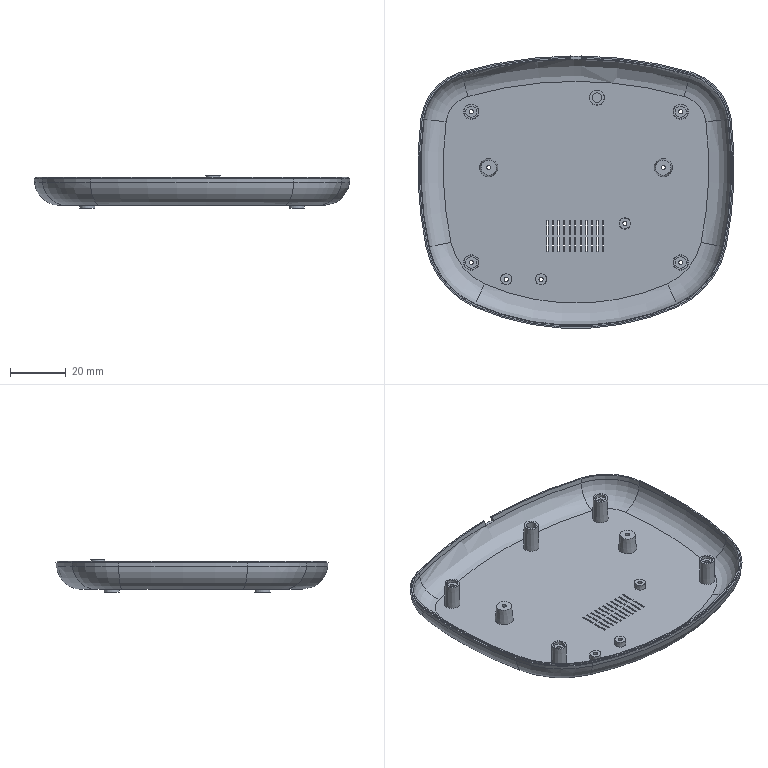Component | NX | XIADIZUO | 1 solid | 193 faces | volume 12367 mm3 | plane 118 | cylinder 31 | cone 28 | torus 16 | commonest cylinder face diameters 1.5 x9 5.5 x4 4 x4 3 x4 299 x2 279 x2 39 x2 59 x2